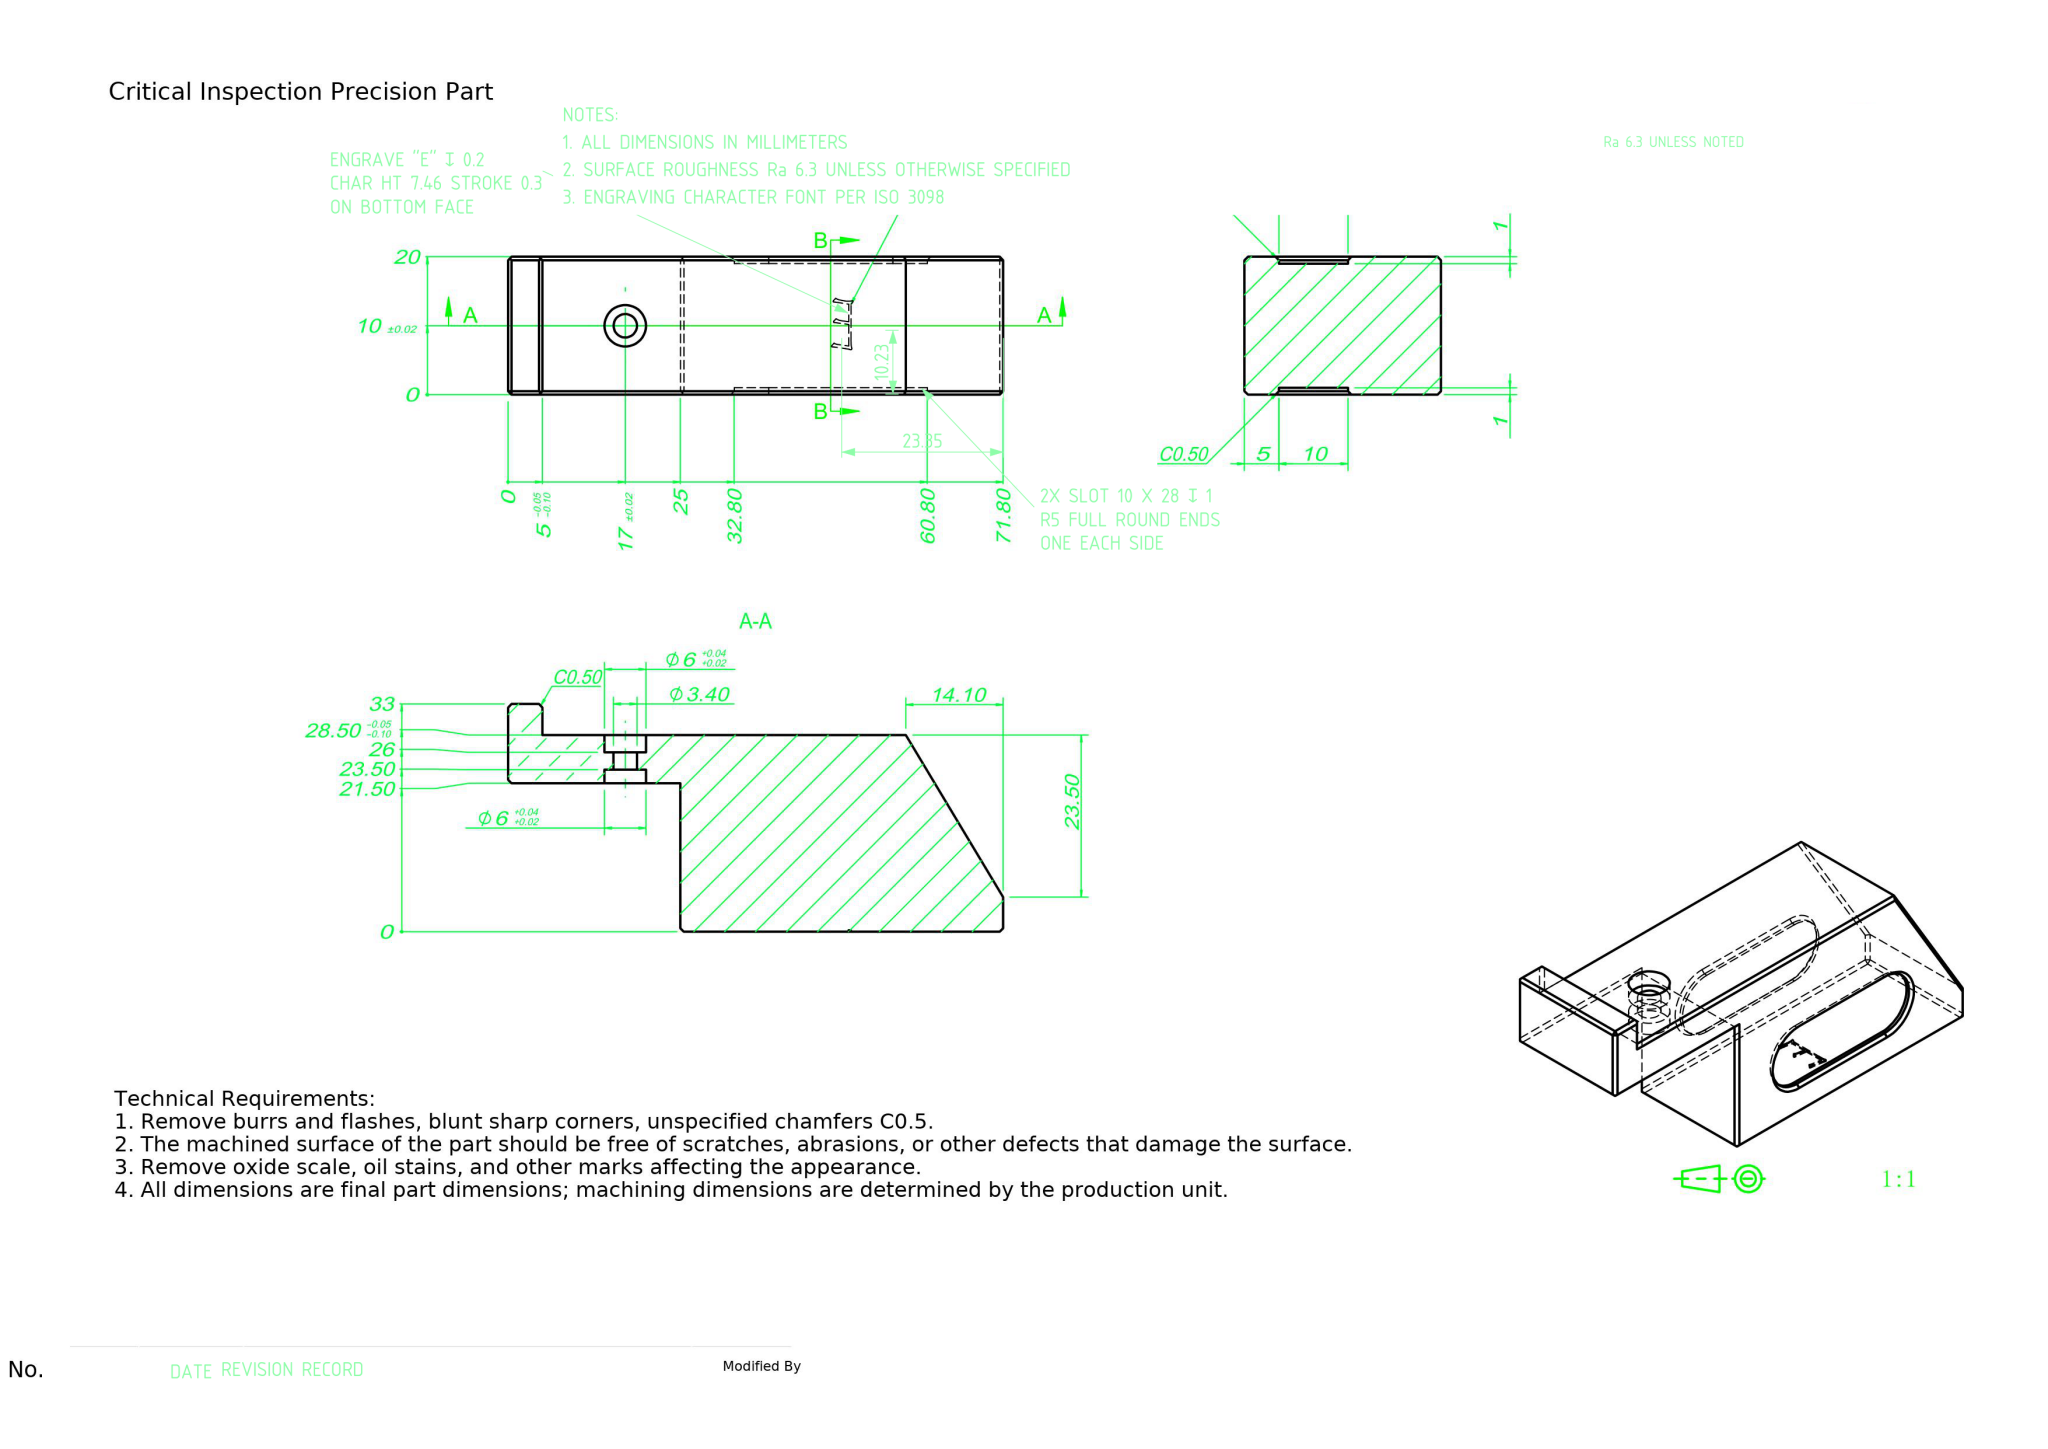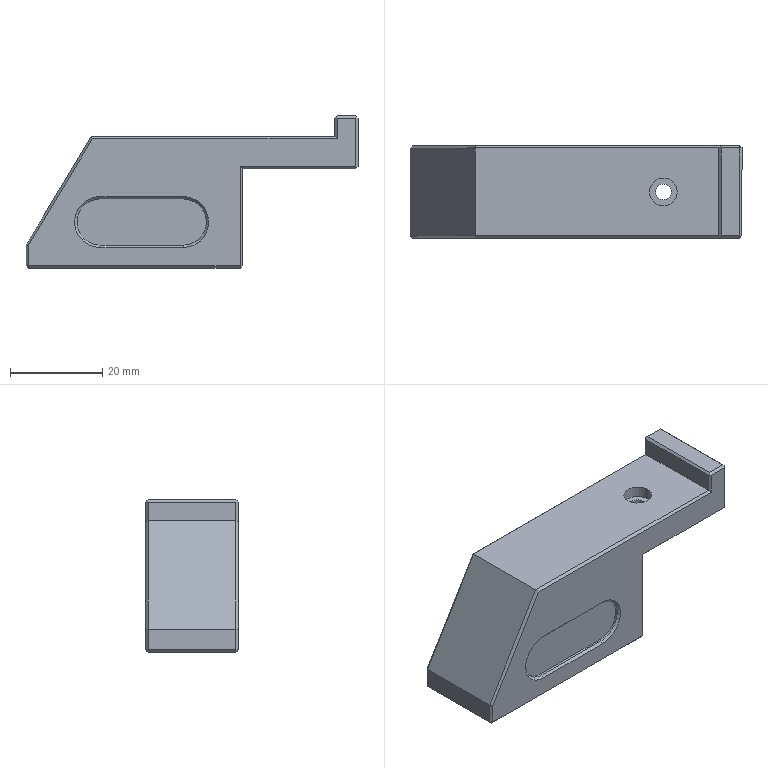Part | NX | mm | 1 solid | 98 faces | box 71.8 x 20 x 33 mm | volume 26566 mm3 | plane 70 | spline 14 | cylinder 10 | cone 4 | commonest cylinder face diameters 6 x4 10 x4 3.4 x2